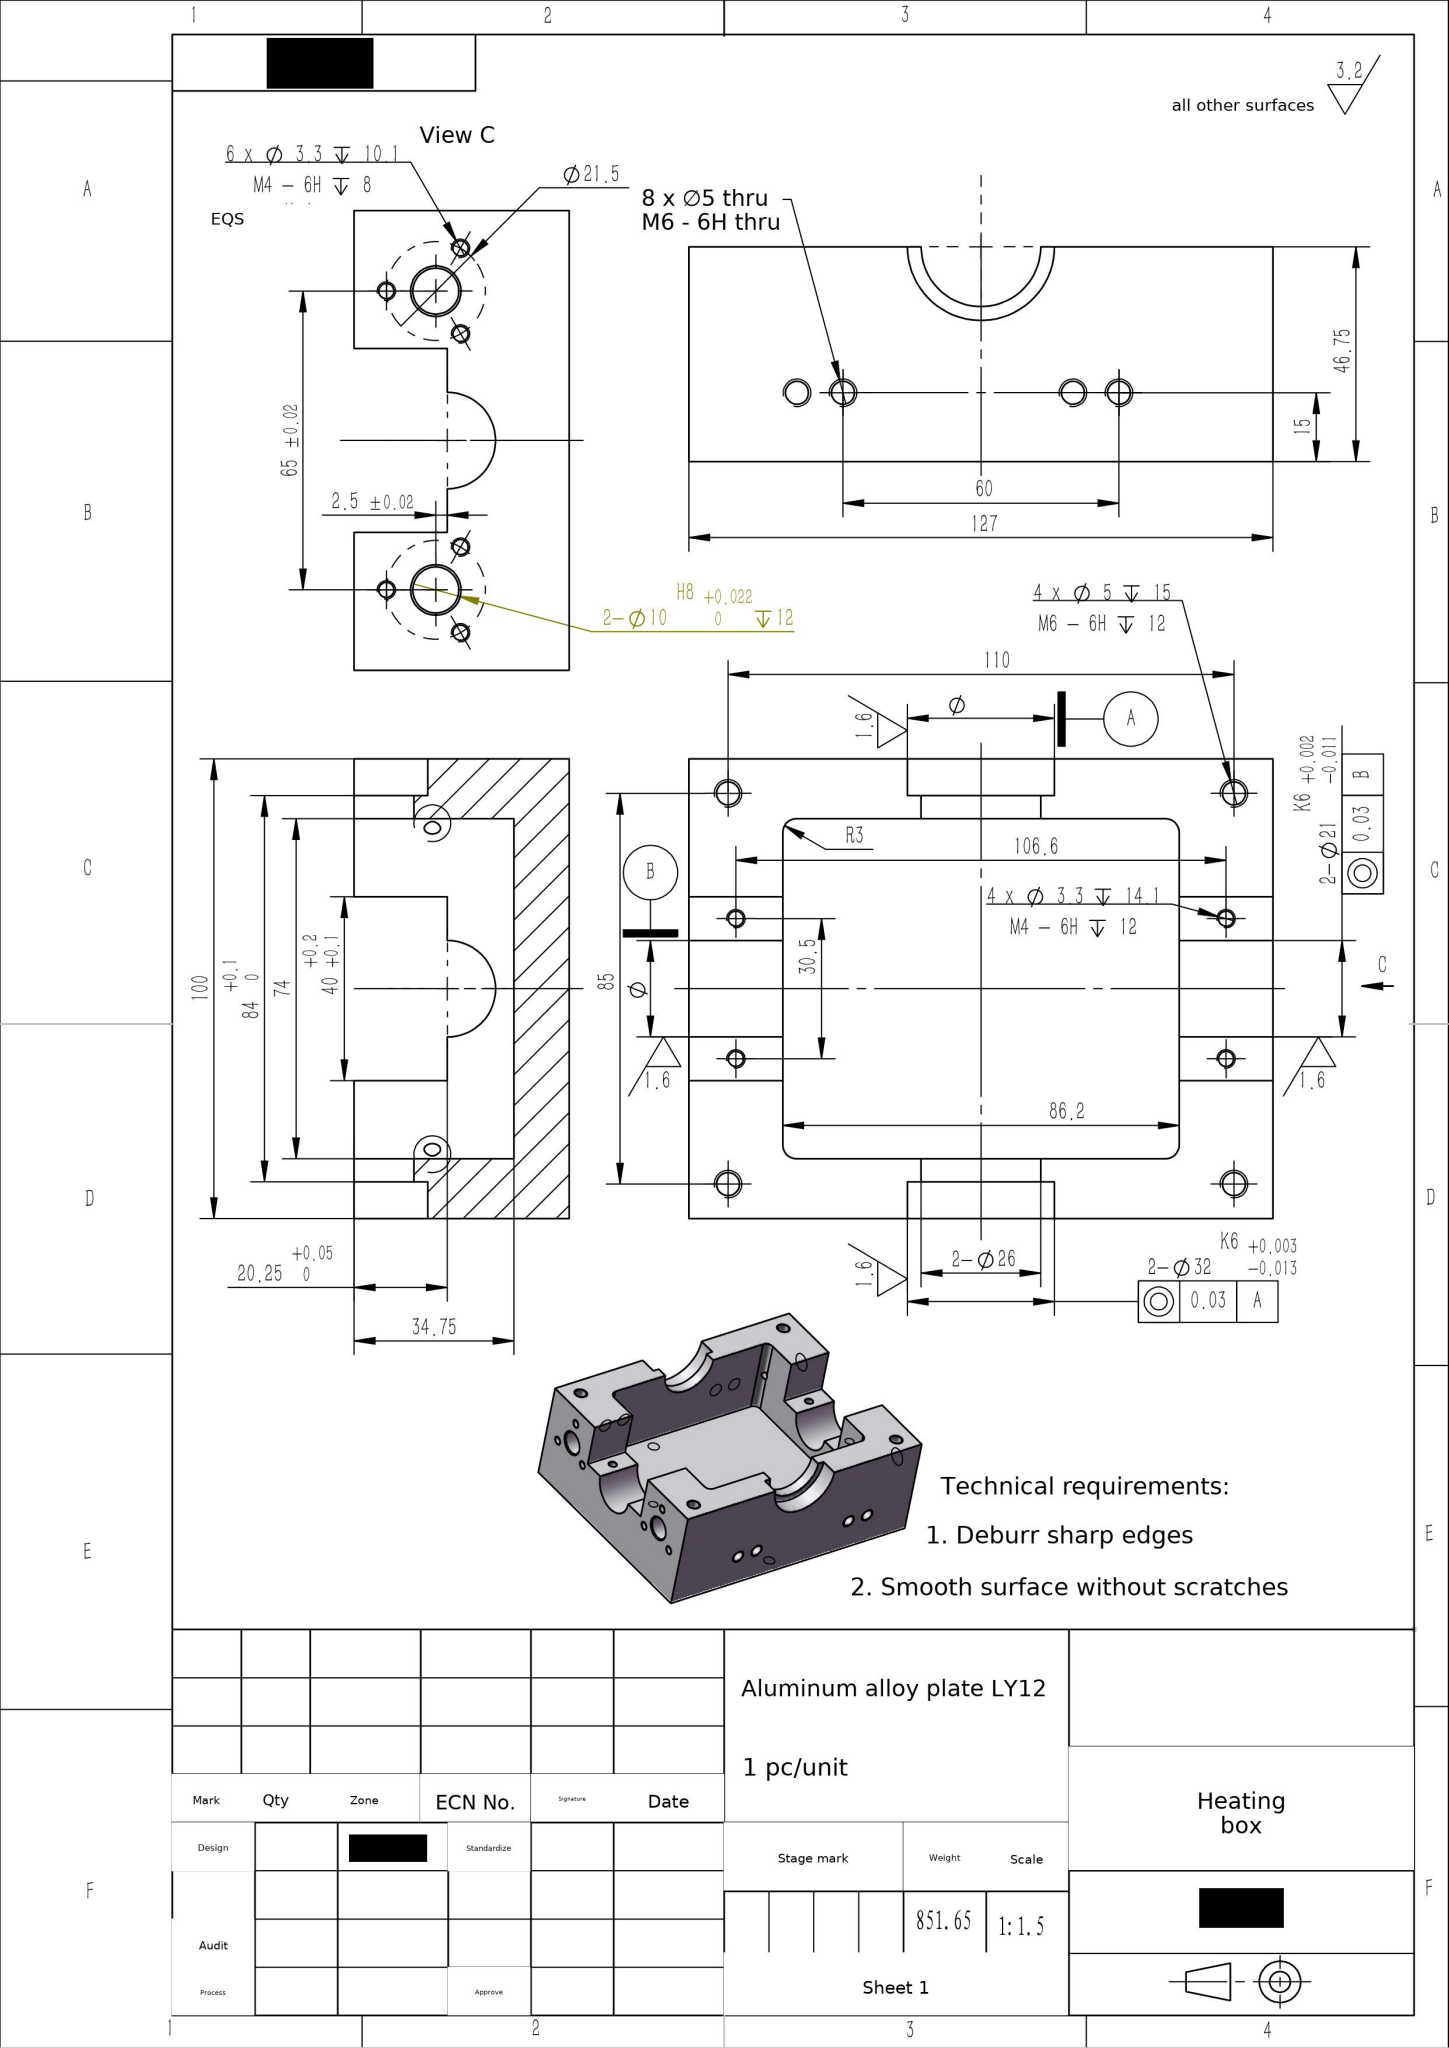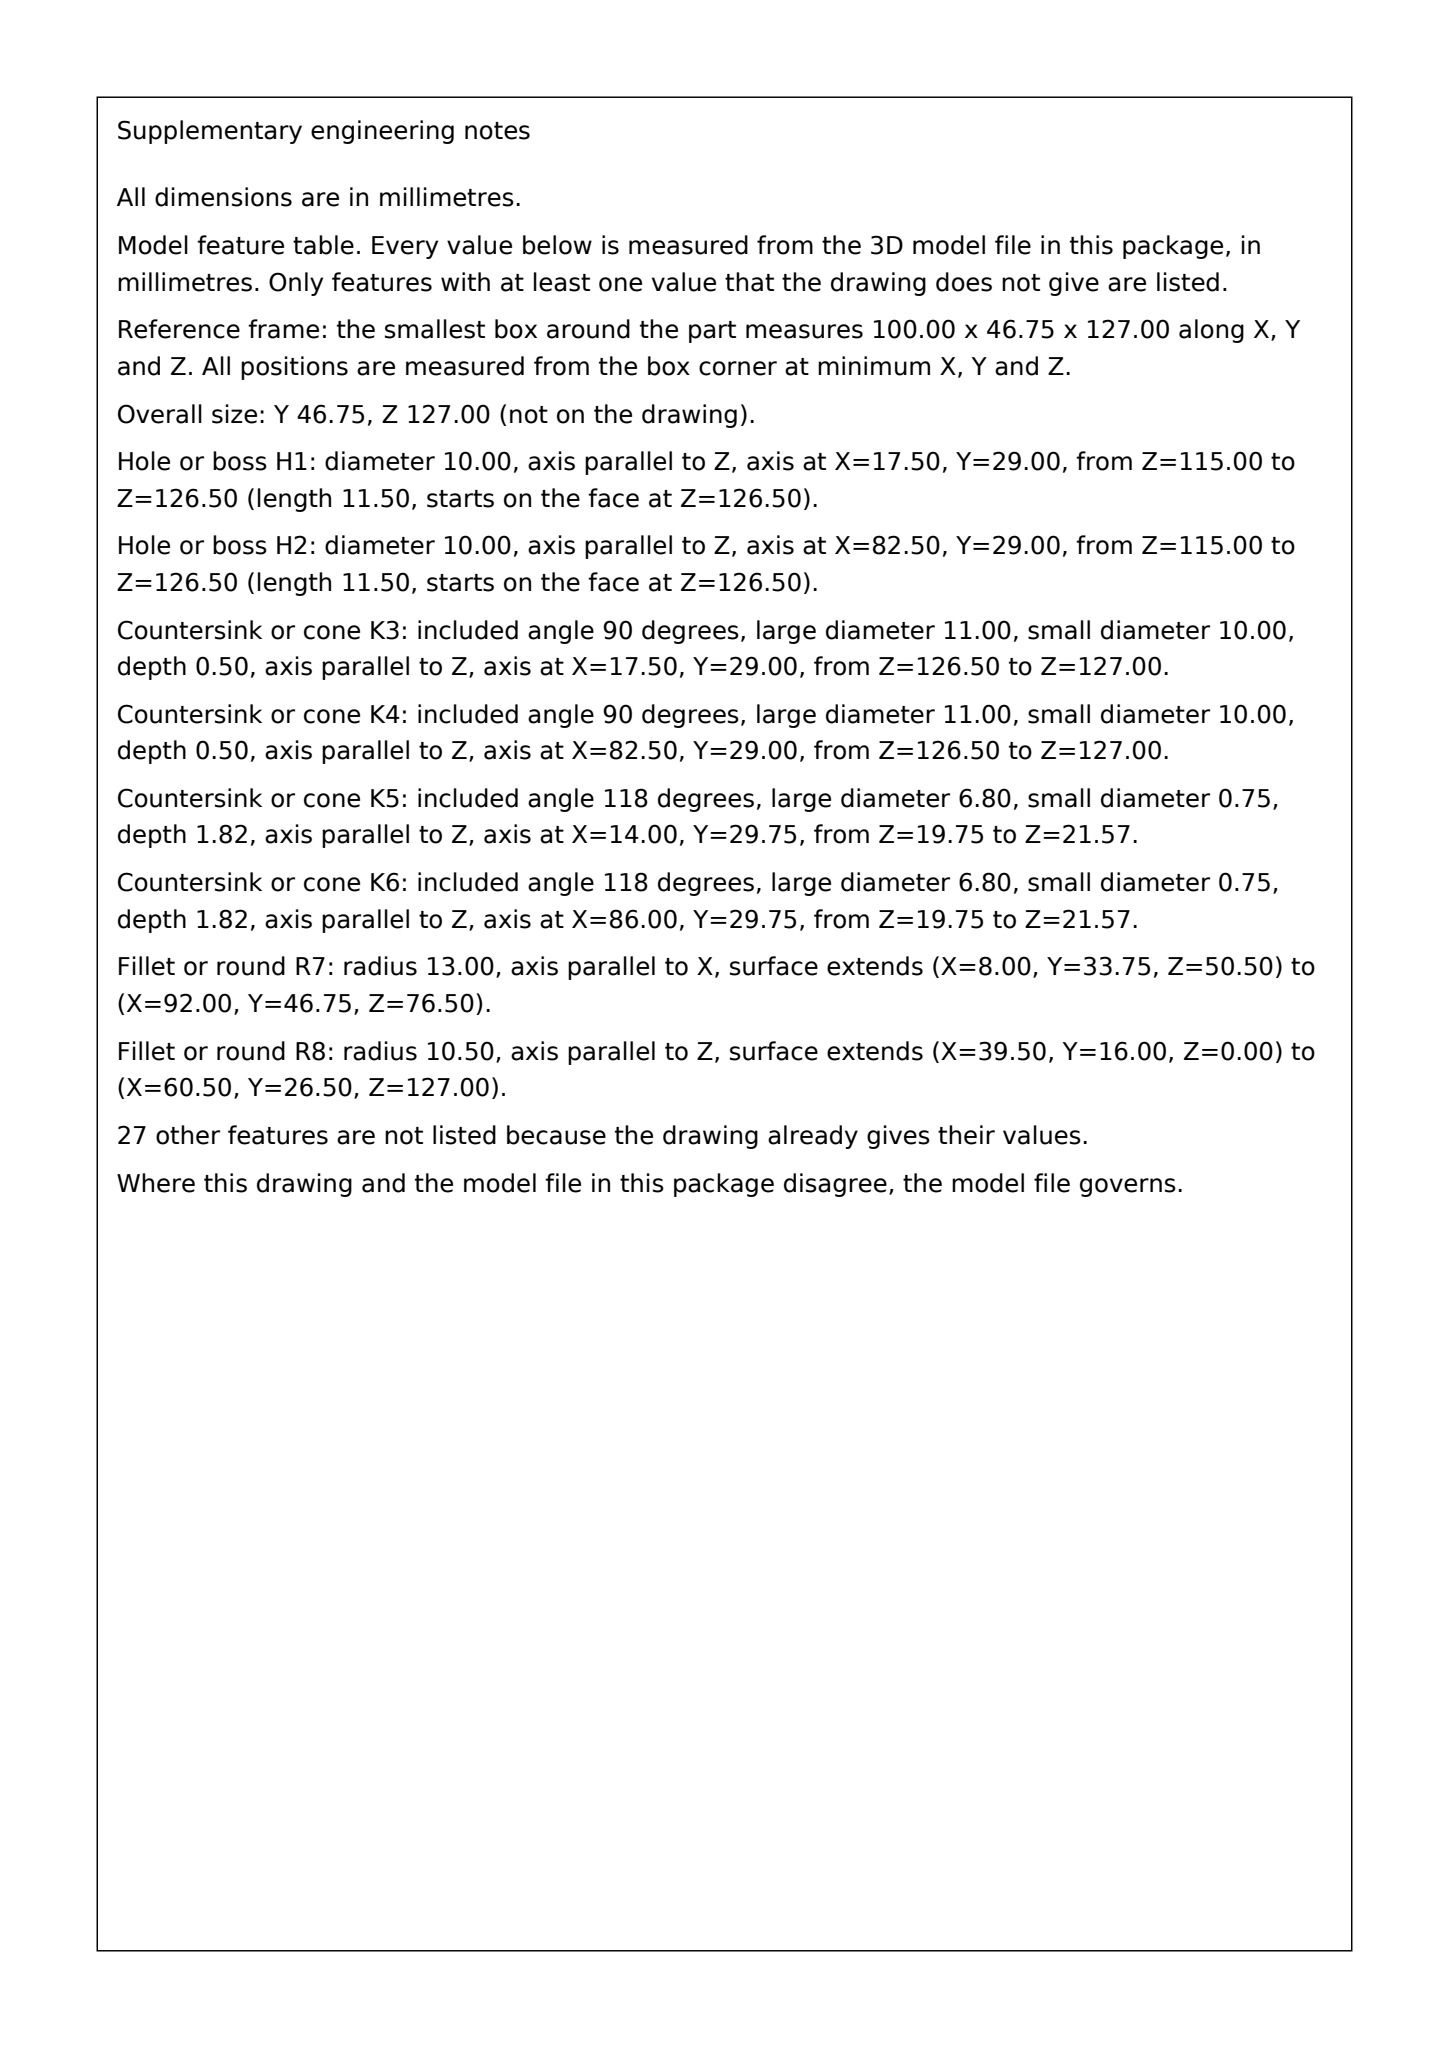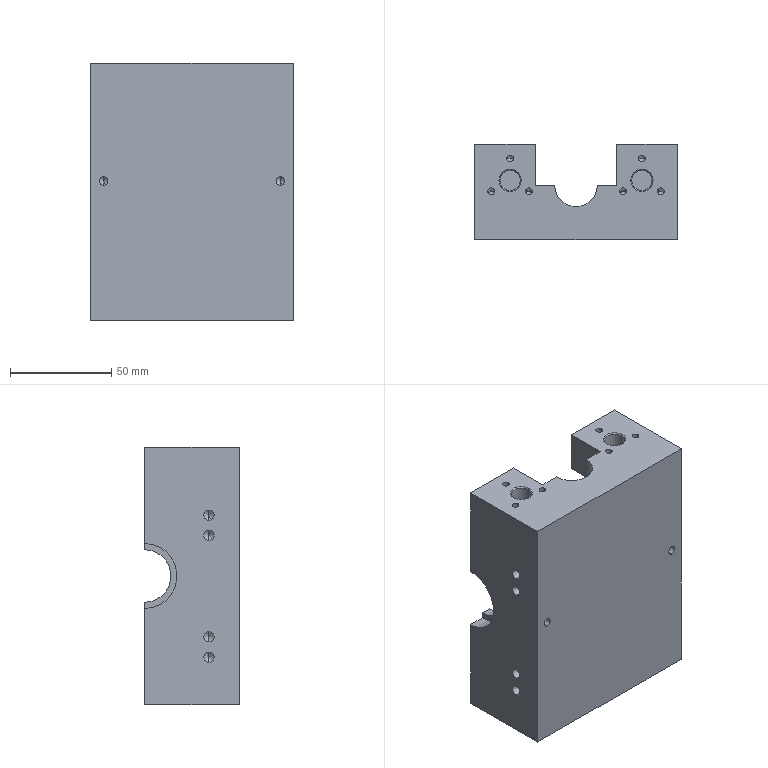Part | SolidWorks | mm | material Aluminum alloy plate LY12 | 1 solid | 148 faces | box 100 x 46.75 x 127 mm | volume 315426 mm3 | cylinder 66 | cone 56 | plane 26 | commonest cylinder face diameters 5 x24 3.3 x20 10 x4 4.2 x4 6.8 x4 6 x4 26 x2 21 x2
build123d program:
from build123d import *

# Parameters (mm, degrees)
SKETCH1_W                  = 100
SKETCH1_H                  = 127
BOSS_EXTRUDE1_DEPTH        = 12
SKETCH2_W                  = 100
SKETCH2_H                  = 127
SKETCH2_W_2                = 74
SKETCH2_H_2                = 86.2
BOSS_EXTRUDE2_DEPTH        = 34.75
F_21_0_21_DIAMETER_HOLE1_D = 21
HOLE1_D                    = 26
SKETCH6_R                  = 16
CUT_EXTRUDE1_DEPTH         = 8
FILLET1_R                  = 3
M6_TAPPED_HOLE1_D          = 5
M6_TAPPED_HOLE1_DEPTH      = 15
M6_TAPPED_HOLE1_TIP        = 1.502
SKETCH11_W                 = 40
SKETCH11_H                 = 20.25
CUT_EXTRUDE2_DEPTH         = 145.273
M4_TAPPED_HOLE1_D          = 3.3
M4_TAPPED_HOLE1_DEPTH      = 14.1
M4_TAPPED_HOLE1_TIP        = 0.9914
M8_TAPPED_HOLE1_D          = 6.8
M8_TAPPED_HOLE1_DEPTH      = 19.75
M8_TAPPED_HOLE1_TIP        = 2.043
M6_TAPPED_HOLE2_AT_2_COUNT = 2
M6_TAPPED_HOLE2_AT_2_PITCH = 60
M5_TAPPED_HOLE1_D          = 4.2
M5_TAPPED_HOLE1_DEPTH      = 12.4
M5_TAPPED_HOLE1_TIP        = 1.262
SKETCH22_R                 = 5
CUT_EXTRUDE3_DEPTH         = 12
CIRPATTERN1_COUNT          = 3
CHAMFER1_SIZE              = 0.5
LPATTERN1_COUNT            = 2
LPATTERN1_PITCH            = 10


with BuildPart() as part:
    # Sketch1 → Boss-Extrude1 (new body)
    with BuildSketch(Plane(origin=(0, 0, 0), x_dir=(1, 0, 0), z_dir=(0, 1, 0))):
        Rectangle(SKETCH1_W, SKETCH1_H)
    extrude(amount=BOSS_EXTRUDE1_DEPTH)

    # Sketch2 → Boss-Extrude2 (add)
    with BuildSketch(Plane(origin=(0, 12, 0), x_dir=(1, 0, 0), z_dir=(0, 1, 0))):
        Rectangle(SKETCH2_W, SKETCH2_H)
        Rectangle(SKETCH2_W_2, SKETCH2_H_2, mode=Mode.SUBTRACT)
    extrude(amount=BOSS_EXTRUDE2_DEPTH)

    # 21.0 _21_ Diameter Hole1 (through all)
    with Locations(Plane.XY.offset(63.5)):
        with Locations((0, 26.5)):
            Hole(F_21_0_21_DIAMETER_HOLE1_D / 2)

    # Hole1 (through all)
    with Locations(Plane(origin=(50, 0, 0), x_dir=(0, 0, -1), z_dir=(1, 0, 0))):
        with Locations((0, 46.75)):
            Hole(HOLE1_D / 2)

    # Sketch6 → Cut-Extrude1 (cut)
    with BuildSketch(Plane(origin=(50, 0, 0), x_dir=(0, 0, -1), z_dir=(1, 0, 0))):
        with Locations((0, 46.75)):
            Circle(SKETCH6_R)
    cut_extrude1 = extrude(amount=-CUT_EXTRUDE1_DEPTH, mode=Mode.SUBTRACT)

    # Mirror1: Cut-Extrude1 across plane
    add(cut_extrude1.mirror(Plane(origin=(0, 0, 0), x_dir=(0, 0, 1), z_dir=(1, 0, 0))), mode=Mode.SUBTRACT)

    # Fillet1
    fillet1_edges = [part.edges().sort_by_distance(p)[0] for p in [
        (-37, 29.375, 43.1),
        (37, 29.375, 43.1),
        (37, 29.375, -43.1),
        (-37, 29.375, -43.1),
    ]]
    fillet(fillet1_edges, radius=FILLET1_R)

    # M6 Tapped Hole1
    with Locations(Plane(origin=(0, 46.75, 0), x_dir=(1, 0, 0), z_dir=(0, 1, 0))):
        with Locations((-42.5, -55), (42.5, -55), (42.5, 55), (-42.5, 55)):
            Hole(M6_TAPPED_HOLE1_D / 2, depth=M6_TAPPED_HOLE1_DEPTH)
            with Locations((0, 0, -(M6_TAPPED_HOLE1_DEPTH + M6_TAPPED_HOLE1_TIP / 2))):  # 118° drill point
                Cone(0, M6_TAPPED_HOLE1_D / 2, M6_TAPPED_HOLE1_TIP, mode=Mode.SUBTRACT)

    # Sketch11 → Cut-Extrude2 (cut, through all)
    with BuildSketch(Plane.XY.offset(63.5)):
        with Locations((0, 36.625)):
            Rectangle(SKETCH11_W, SKETCH11_H)
    extrude(amount=-CUT_EXTRUDE2_DEPTH, mode=Mode.SUBTRACT)

    # M4 Tapped Hole1
    with Locations(Plane(origin=(0, 26.5, 0), x_dir=(1, 0, 0), z_dir=(0, 1, 0))):
        with Locations((-15.25, -53.3), (15.25, -53.3), (-15.25, 53.3), (15.25, 53.3)):
            Hole(M4_TAPPED_HOLE1_D / 2, depth=M4_TAPPED_HOLE1_DEPTH)
            with Locations((0, 0, -(M4_TAPPED_HOLE1_DEPTH + M4_TAPPED_HOLE1_TIP / 2))):  # 118° drill point
                Cone(0, M4_TAPPED_HOLE1_D / 2, M4_TAPPED_HOLE1_TIP, mode=Mode.SUBTRACT)

    # M8 Tapped Hole1
    with Locations(Plane(origin=(0, 0, -63.5), x_dir=(-1, 0, 0), z_dir=(0, 0, -1))):
        with Locations((-36, 29.75), (36, 29.75)):
            Hole(M8_TAPPED_HOLE1_D / 2, depth=M8_TAPPED_HOLE1_DEPTH)
            with Locations((0, 0, -(M8_TAPPED_HOLE1_DEPTH + M8_TAPPED_HOLE1_TIP / 2))):  # 118° drill point
                Cone(0, M8_TAPPED_HOLE1_D / 2, M8_TAPPED_HOLE1_TIP, mode=Mode.SUBTRACT)

    # Sketch17 → M6 Tapped Hole2 (revolve, cut)
    with BuildSketch(Plane(origin=(-50, 15, -30), x_dir=(0, 0, 1), z_dir=(0, 1, 0))):
        Polygon((0, 0), (0, 12.002), (2.5, 10.5), (2.5, 0), align=None)
    m6_tapped_hole2 = revolve(axis=Axis((-56.35, 15, -30), (1, 0, 0)), mode=Mode.SUBTRACT)

    # M6 Tapped Hole2 at 2: M6 Tapped Hole2 ×2
    with Locations(*[(0, 0, i * M6_TAPPED_HOLE2_AT_2_PITCH) for i in range(1, M6_TAPPED_HOLE2_AT_2_COUNT)]):
        add(m6_tapped_hole2, mode=Mode.SUBTRACT)

    # Mirror2: M6 Tapped Hole2 across plane
    add(m6_tapped_hole2.mirror(Plane(origin=(0, 0, 0), x_dir=(0, 0, 1), z_dir=(1, 0, 0))), mode=Mode.SUBTRACT)

    # Mirror2 copy 1 sketch → Mirror2 copy 1 (revolve, cut)
    with BuildSketch(Plane(origin=(50, 15, 30), x_dir=(0, 0, 1), z_dir=(0, 1, 0))):
        Polygon((0, 0), (0, -12.002), (2.5, -10.5), (2.5, 0), align=None)
    revolve(axis=Axis((56.35, 15, 30), (1, 0, 0)), mode=Mode.SUBTRACT)

    # M5 Tapped Hole1
    with Locations(Plane(origin=(0, 0, 0), x_dir=(-1, 0, 0), z_dir=(0, -1, 0))):
        with Locations((-43.5, -5.475), (43.5, -5.475)):
            Hole(M5_TAPPED_HOLE1_D / 2, depth=M5_TAPPED_HOLE1_DEPTH)
            with Locations((0, 0, -(M5_TAPPED_HOLE1_DEPTH + M5_TAPPED_HOLE1_TIP / 2))):  # 118° drill point
                Cone(0, M5_TAPPED_HOLE1_D / 2, M5_TAPPED_HOLE1_TIP, mode=Mode.SUBTRACT)

    # Sketch22 → Cut-Extrude3 (cut)
    with BuildSketch(Plane.XY.offset(63.5)):
        with Locations((-32.5, 29)):
            Circle(SKETCH22_R)
        with Locations(Location((32.5, 29, 0), (0, 0, 180))):
            Circle(SKETCH22_R)
    extrude(amount=-CUT_EXTRUDE3_DEPTH, mode=Mode.SUBTRACT)

    # Sketch24 → M4 Tapped Hole2 (revolve, cut)
    with BuildSketch(Plane(origin=(-32.5, 39.75, 63.5), x_dir=(0, -1, 0), z_dir=(1, 0, 0))):
        Polygon((0, 0), (0, 11.091), (1.65, 10.1), (1.65, 0), align=None)
    m4_tapped_hole2 = revolve(axis=Axis((-32.5, 39.75, 69.85), (0, 0, -1)), mode=Mode.SUBTRACT)

    # CirPattern1: M4 Tapped Hole2 ×3 about axis
    cirpattern1_axis = Axis((-32.5, 29, 0), (0, 0, 1))
    for i in range(1, CIRPATTERN1_COUNT):
        add(m4_tapped_hole2.rotate(cirpattern1_axis, i * 360 / CIRPATTERN1_COUNT), mode=Mode.SUBTRACT)

    # Mirror3: M4 Tapped Hole2 across plane
    add(m4_tapped_hole2.mirror(Plane(origin=(0, 0, 0), x_dir=(0, 0, 1), z_dir=(1, 0, 0))), mode=Mode.SUBTRACT)

    # Mirror3 copy 1 sketch → Mirror3 copy 1 (revolve, cut)
    with BuildSketch(Plane(origin=(41.81, 23.625, 63.5), x_dir=(-0.866, 0.5, 0), z_dir=(0.5, 0.866, 0))):
        Polygon((0, 0), (0, -11.091), (1.65, -10.1), (1.65, 0), align=None)
    revolve(axis=Axis((41.81, 23.625, 69.85), (0, 0, 1)), mode=Mode.SUBTRACT)

    # Mirror3 copy 2 sketch → Mirror3 copy 2 (revolve, cut)
    with BuildSketch(Plane(origin=(23.19, 23.625, 63.5), x_dir=(0.866, 0.5, 0), z_dir=(0.5, -0.866, 0))):
        Polygon((0, 0), (0, -11.091), (1.65, -10.1), (1.65, 0), align=None)
    revolve(axis=Axis((23.19, 23.625, 69.85), (0, 0, 1)), mode=Mode.SUBTRACT)

    # Chamfer1
    chamfer1_edges = [part.edges().sort_by_distance(p)[0] for p in [
        (-37.5, 29, 63.5),
        (37.5, 29, 63.5),
    ]]
    chamfer(chamfer1_edges, length=CHAMFER1_SIZE)

    # LPattern1: M6 Tapped Hole2 ×2
    with Locations(*[(0, 0, -i * LPATTERN1_PITCH) for i in range(1, LPATTERN1_COUNT)]):
        add(m6_tapped_hole2, mode=Mode.SUBTRACT)

    # LPattern1 copy 1 sketch → LPattern1 copy 1 (revolve, cut)
    with BuildSketch(Plane(origin=(-50, 15, 20), x_dir=(0, 0, 1), z_dir=(0, 1, 0))):
        Polygon((0, 0), (0, 12.002), (2.5, 10.5), (2.5, 0), align=None)
    revolve(axis=Axis((-56.35, 15, 20), (1, 0, 0)), mode=Mode.SUBTRACT)

    # LPattern1 copy 2 sketch → LPattern1 copy 2 (revolve, cut)
    with BuildSketch(Plane(origin=(50, 15, -40), x_dir=(0, 0, 1), z_dir=(0, 1, 0))):
        Polygon((0, 0), (0, -12.002), (2.5, -10.5), (2.5, 0), align=None)
    revolve(axis=Axis((56.35, 15, -40), (1, 0, 0)), mode=Mode.SUBTRACT)

    # LPattern1 copy 3 sketch → LPattern1 copy 3 (revolve, cut)
    with BuildSketch(Plane(origin=(50, 15, 20), x_dir=(0, 0, 1), z_dir=(0, 1, 0))):
        Polygon((0, 0), (0, -12.002), (2.5, -10.5), (2.5, 0), align=None)
    revolve(axis=Axis((56.35, 15, 20), (1, 0, 0)), mode=Mode.SUBTRACT)


solid = part.part